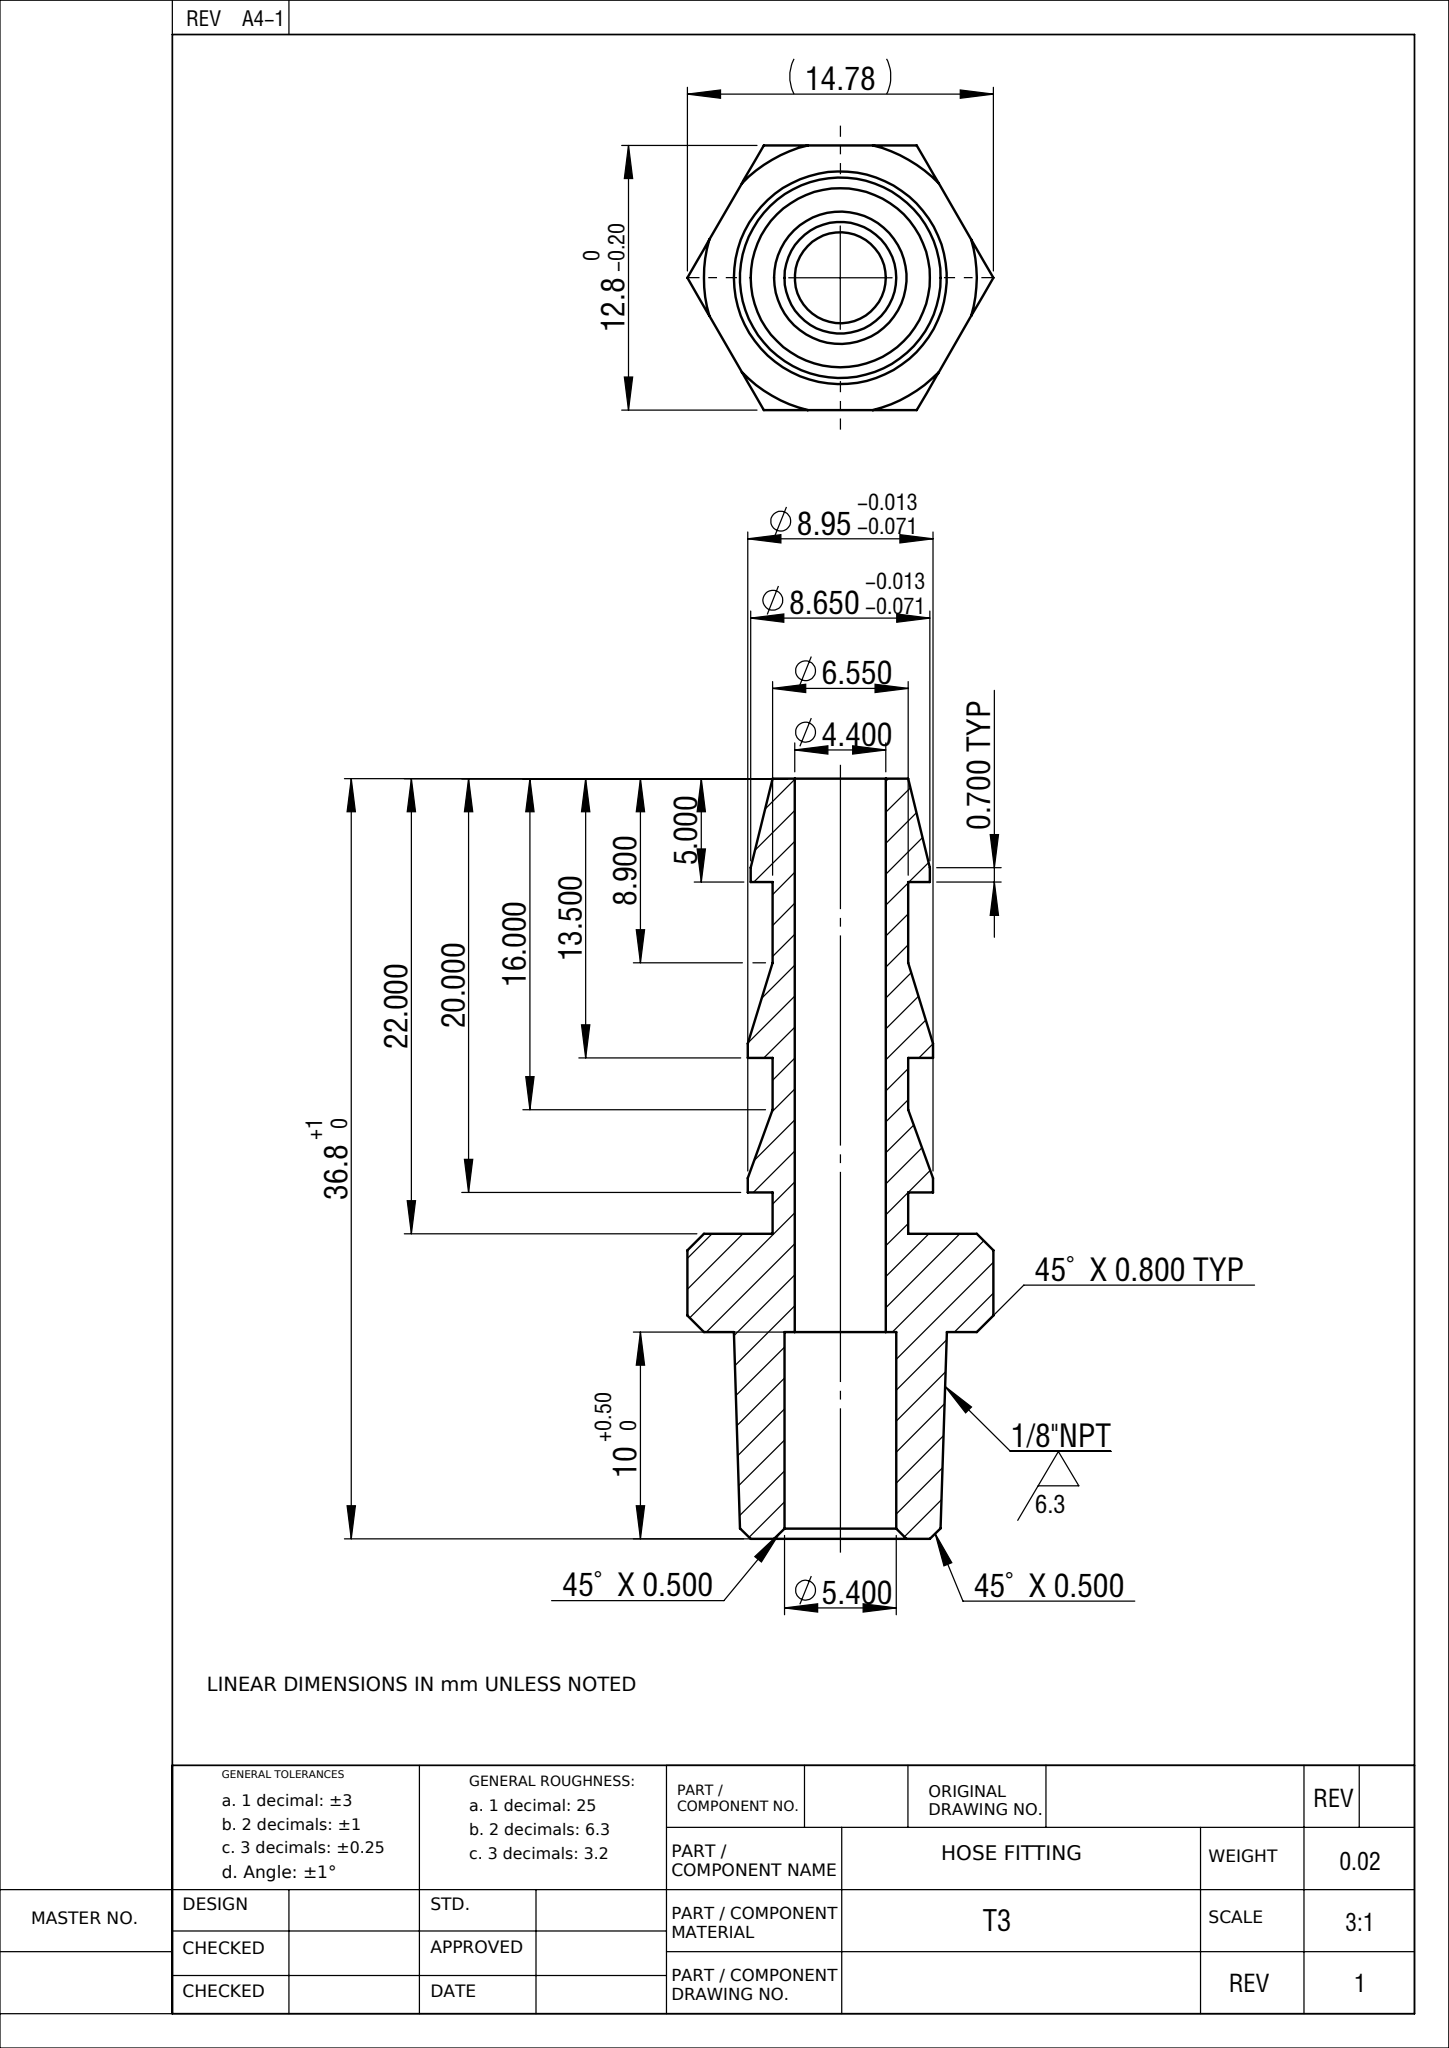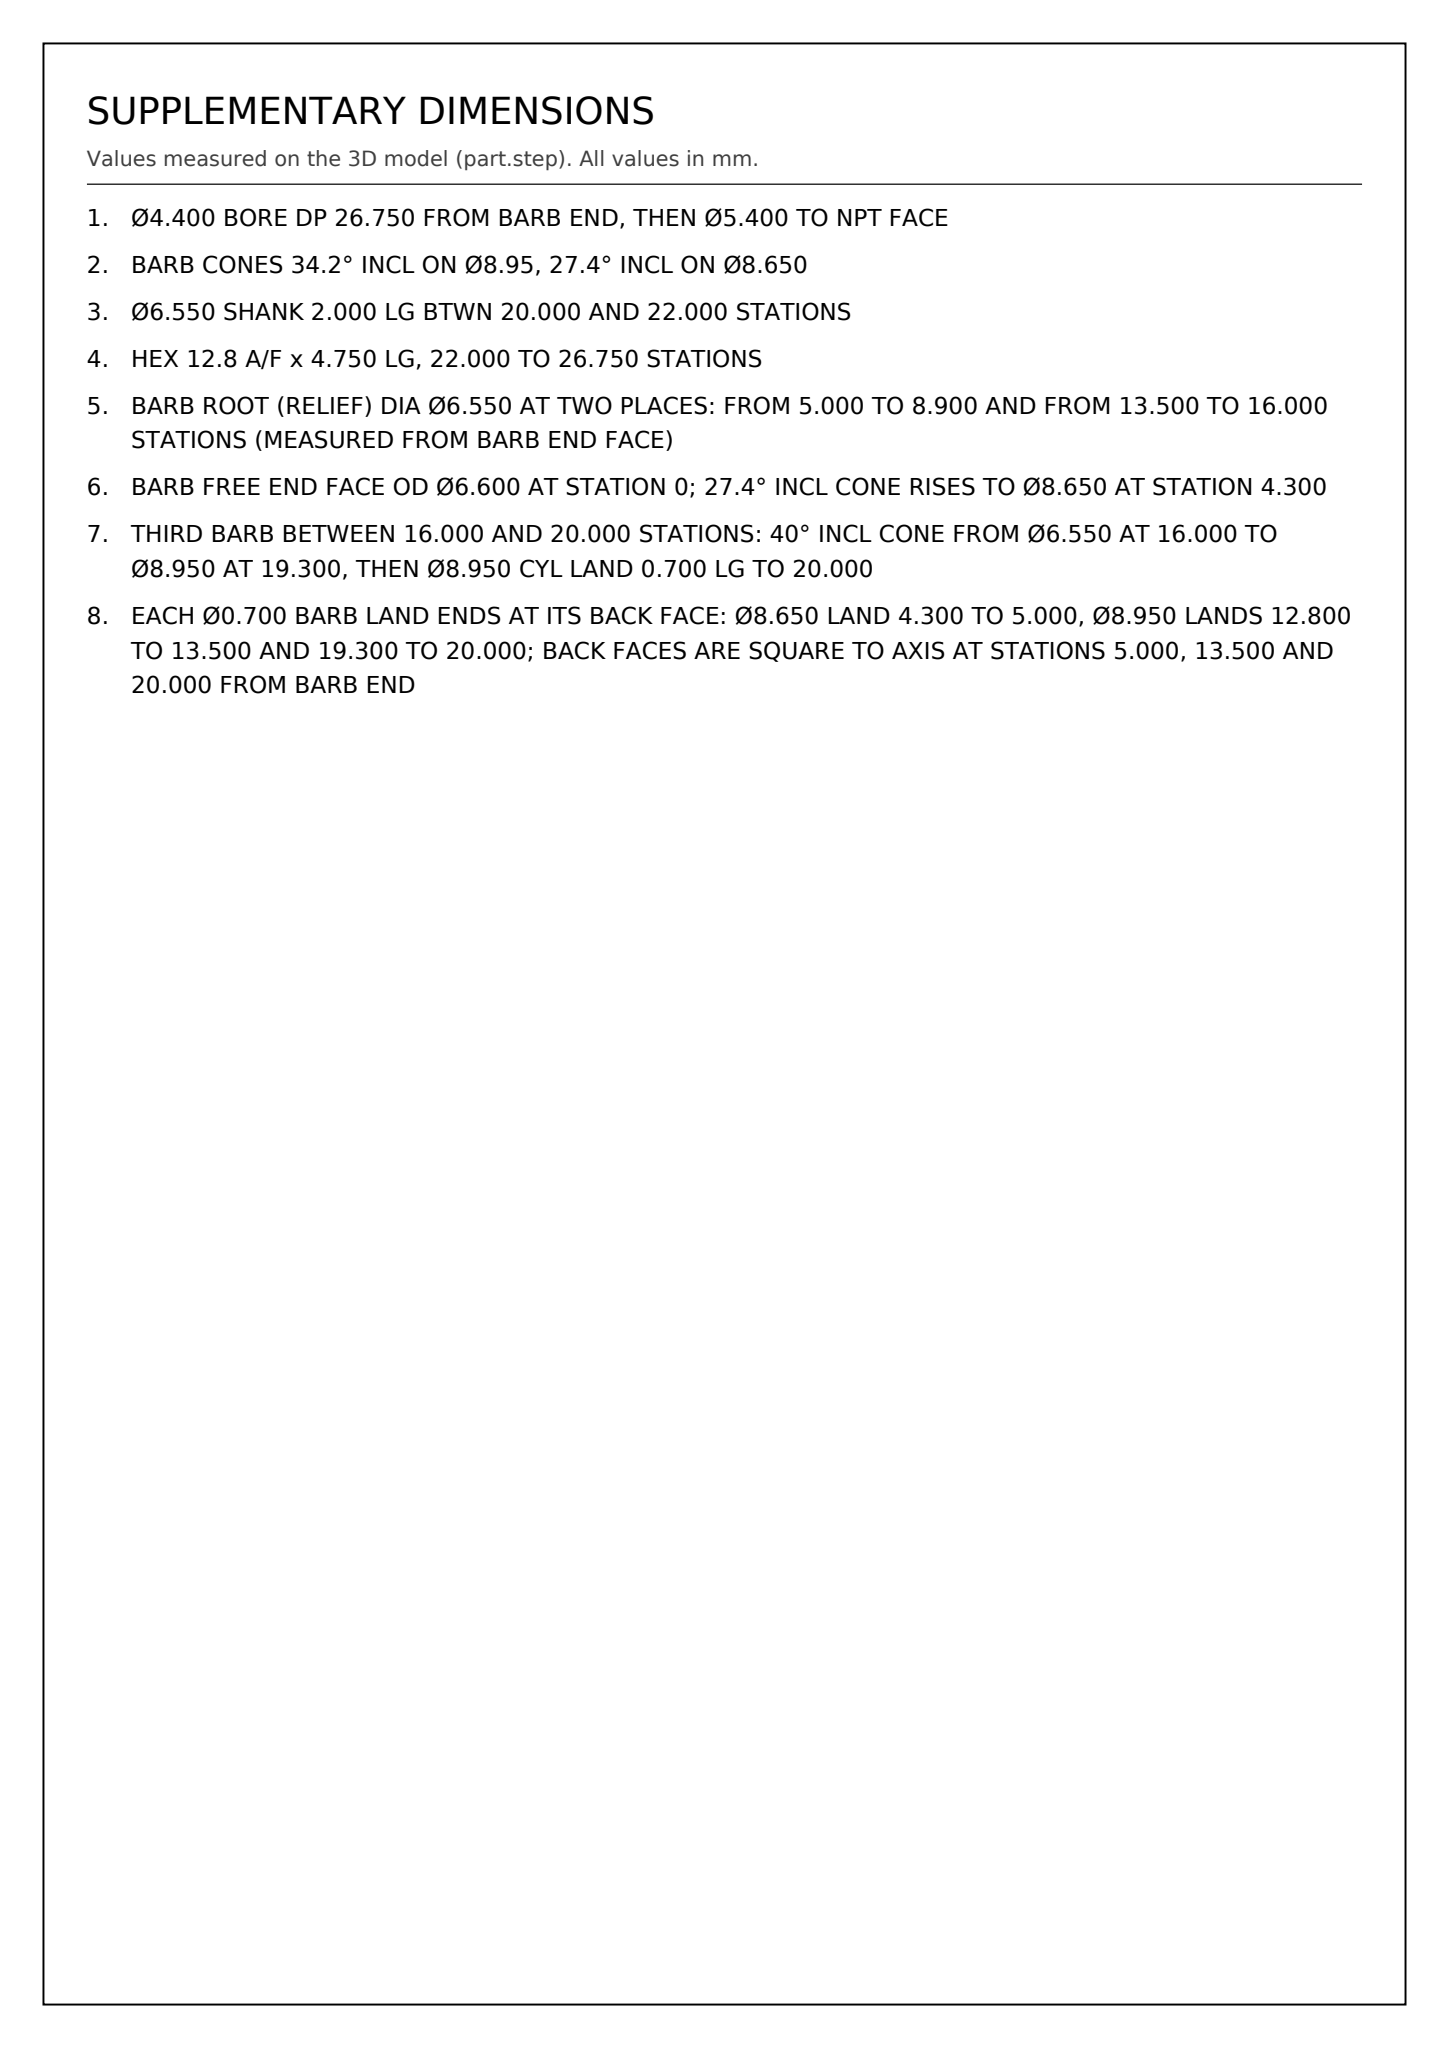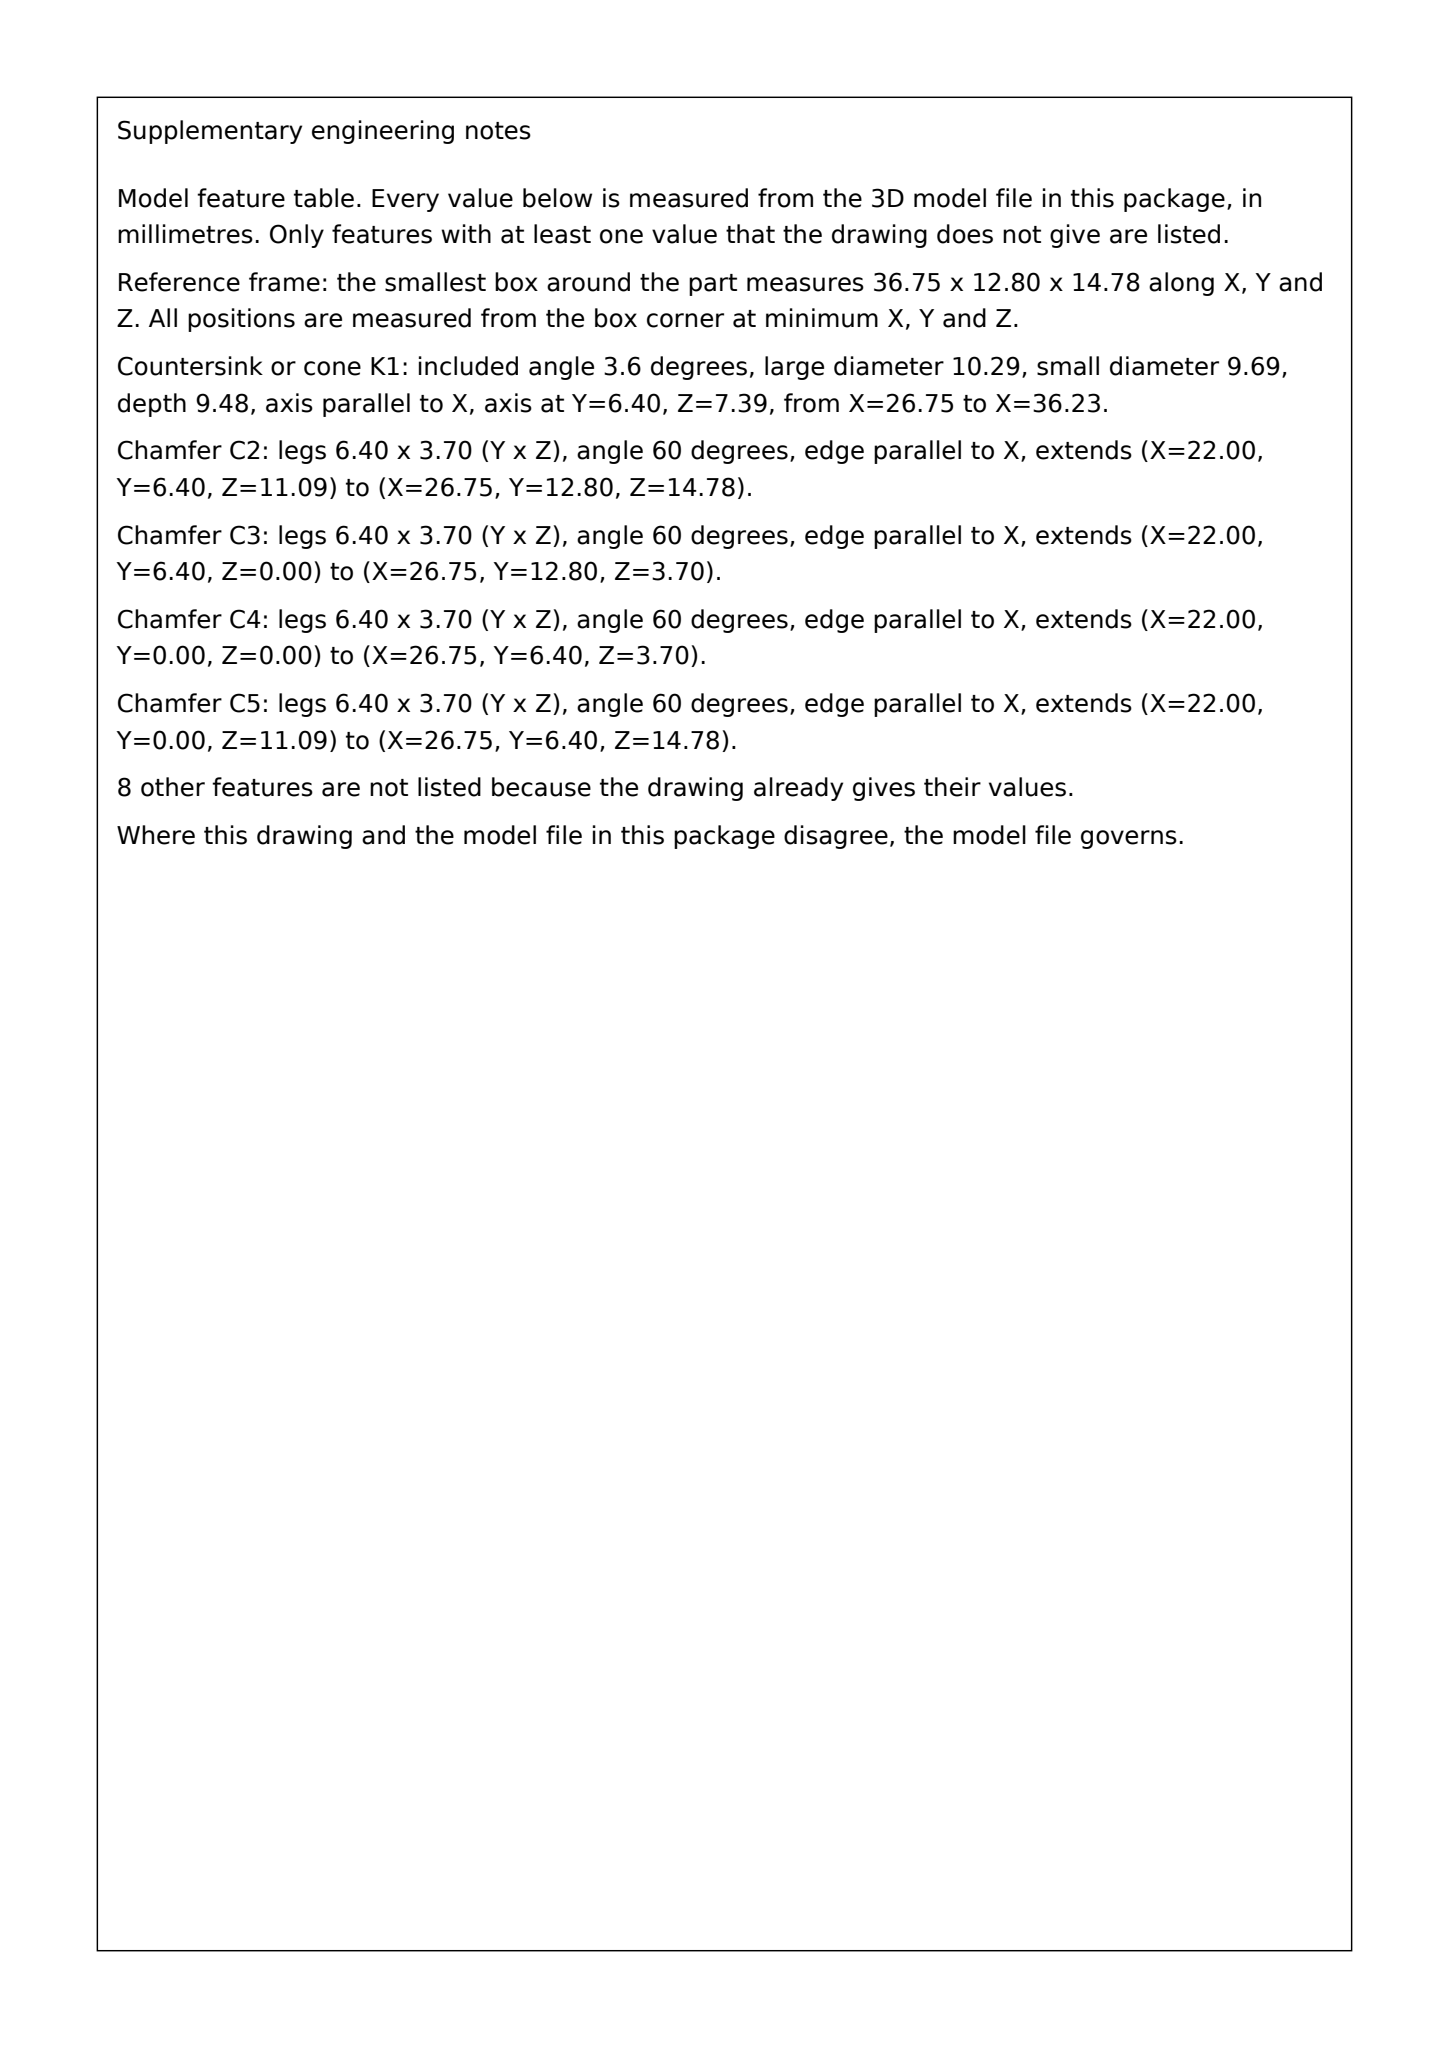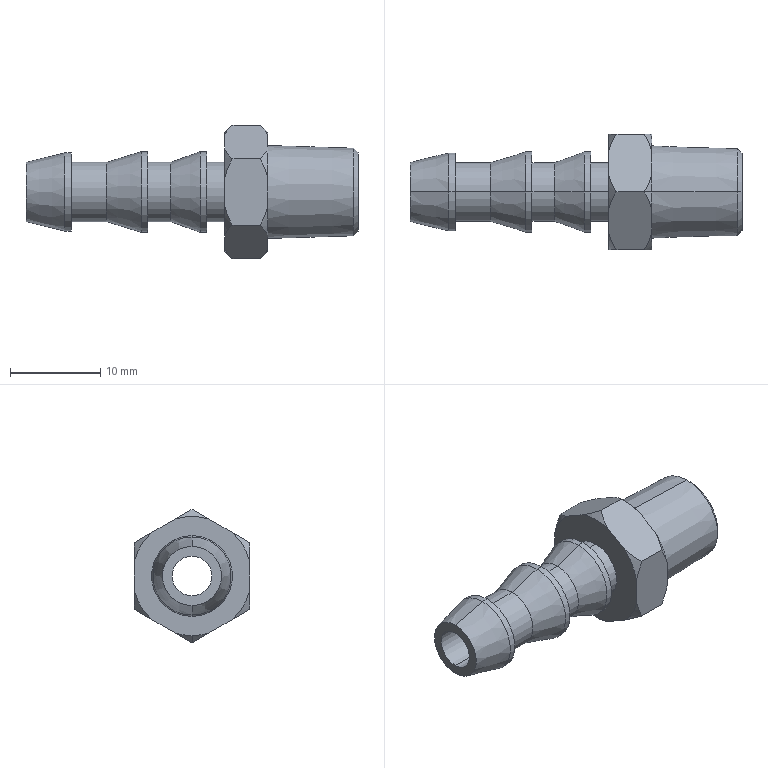Part | SolidWorks | mm | 1 solid | 56 faces | box 36.75 x 12.8 x 14.78 mm | volume 1761 mm3 | cone 26 | cylinder 16 | plane 14 | commonest cylinder face diameters 6.55 x6 8.95 x4 5.4 x2 8.65 x2 4.4 x2
Drawing notes:
Ø4.400 BORE DP 26.750 FROM BARB END, THEN Ø5.400 TO NPT FACE | from the solid: Ø4.4 cyl L=26.75 from x=0; Ø5.4 cyl L=9.5 from x=26.75 to 36.25; bbox L=36.75
BARB CONES 34.2° INCL ON Ø8.95, 27.4° INCL ON Ø8.650 | from the solid: cones [34.2, ref_dia 8.95] and [27.4, ref_dia 8.65]
Ø6.550 SHANK 2.000 LG BTWN 20.000 AND 22.000 STATIONS | from the solid: Ø6.55 cylinder L=2.0 between axis planes x=20.0 and x=22.0
HEX 12.8 A/F x 4.750 LG, 22.000 TO 26.750 STATIONS | from the solid: axis planes x=22.0 and x=26.75; 26.75 = 36.75 - 10 NPT length
BARB ROOT (RELIEF) DIA Ø6.550 AT TWO PLACES: FROM 5.000 TO 8.900 AND FROM 13.500 TO 16.000 STATIONS (MEASURED FROM BARB END FACE) | from the solid: cylinders: boss/shaft Ø6.55 x from 5.0 to 8.9; boss/shaft Ø6.55 x from 13.5 to 16.0
BARB FREE END FACE OD Ø6.600 AT STATION 0; 27.4° INCL CONE RISES TO Ø8.650 AT STATION 4.300 | from the solid: axis plane x=0.0 extent y [3.9,10.5] / z [4.1,10.7] = 6.6 annulus OD; cone 27.4° ref dia 8.65 from x 0.0, length 4.3
THIRD BARB BETWEEN 16.000 AND 20.000 STATIONS: 40° INCL CONE FROM Ø6.550 AT 16.000 TO Ø8.950 AT 19.300, THEN Ø8.950 CYL LAND 0.700 LG TO 20.000 | from the solid: cone 40.0° ref dia 8.95 bbox_from x=16.0 size x 3.3; cylinder boss/shaft Ø8.95 x from 19.3 to 20.0
EACH Ø0.700 BARB LAND ENDS AT ITS BACK FACE: Ø8.650 LAND 4.300 TO 5.000, Ø8.950 LANDS 12.800 TO 13.500 AND 19.300 TO 20.000; BACK FACES ARE SQUARE TO AXIS AT STATIONS 5.000, 13.500 AND 20.000 FROM BARB END | from the solid: cylinders Ø8.65 x 4.3-5.0, Ø8.95 x 12.8-13.5, Ø8.95 x 19.3-20.0; axis planes x=5.0, x=13.5, x=20.0
build123d program:
from build123d import *
from OCP.BRepFilletAPI import BRepFilletAPI_MakeChamfer

# Parameters (mm, degrees)
CUT_EXTRUDE1_REACH = 40.207
SKETCH2_R          = 2.2
CUT_EXTRUDE2_START = -6
CUT_EXTRUDE2_DEPTH = 6
SKETCH4_R          = 2.7
CUT_EXTRUDE3_DEPTH = 10
CHAMFER1_SIZE      = 0.5
CHAMFER1_SIZE2     = 0.5164


with BuildPart() as part:
    # Sketch1 → Revolve1 (revolve)
    with BuildSketch(Plane.XY, mode=Mode.PRIVATE) as revolve1_sk:
        Polygon((-27.85, 3.275), (-31.75, 3.275), (-31.75, 4.325), (-32.45, 4.325), (-36.75, 3.275), (-36.75, 0), (0, 0), (0, 4.831), (-10, 5.144), (-10, 7.39), (-14.75, 7.39), (-14.75, 3.275), (-16.75, 3.275), (-16.75, 4.475), (-17.45, 4.475), (-20.75, 3.275), (-23.25, 3.275), (-23.25, 4.475), (-23.95, 4.475), align=None)
    revolve(revolve1_sk.sketch.rotate(Axis((-78.266, 0, 0), (1, 0, 0)), 90), axis=Axis((-78.266, 0, 0), (1, 0, 0)))

    # Sketch2 → Cut-Extrude1 (cut, up to next)
    with BuildSketch(Plane(origin=(0, 0, 0), x_dir=(0, 0, -1), z_dir=(1, 0, 0)), mode=Mode.PRIVATE) as cut_extrude1_sk1:
        Circle(SKETCH2_R)
    cut_extrude1_tool1 = extrude(cut_extrude1_sk1.sketch, amount=-CUT_EXTRUDE1_REACH, mode=Mode.PRIVATE) & part.part
    add(cut_extrude1_tool1.solids().sort_by_distance((0, 0, 0))[0], mode=Mode.SUBTRACT)

    # Sketch3 → Cut-Extrude2 (cut)
    with BuildSketch(Plane(origin=(-10, 0, 0), x_dir=(0, 0, -1), z_dir=(1, 0, 0)).offset(CUT_EXTRUDE2_START)):
        with BuildLine():
            Line((-7.39, 0), (-3.695, 6.4))
            ThreePointArc((-3.695, 6.4), (-6.4, 3.695), (-7.39, 0))
        make_face()
        with BuildLine():
            ThreePointArc((3.695, 6.4), (0, 7.39), (-3.695, 6.4))
            Line((-3.695, 6.4), (3.695, 6.4))
        make_face()
        with BuildLine():
            ThreePointArc((7.39, 0), (6.4, 3.695), (3.695, 6.4))
            Line((3.695, 6.4), (7.39, 0))
        make_face()
        with BuildLine():
            ThreePointArc((3.695, -6.4), (6.4, -3.695), (7.39, 0))
            Line((7.39, 0), (3.695, -6.4))
        make_face()
        with BuildLine():
            Line((3.695, -6.4), (-3.695, -6.4))
            ThreePointArc((-3.695, -6.4), (0, -7.39), (3.695, -6.4))
        make_face()
        with BuildLine():
            Line((-3.695, -6.4), (-7.39, 0))
            ThreePointArc((-7.39, 0), (-6.4, -3.695), (-3.695, -6.4))
        make_face()
    extrude(amount=CUT_EXTRUDE2_DEPTH, mode=Mode.SUBTRACT)

    # Sketch4 → Cut-Extrude3 (cut)
    with BuildSketch(Plane(origin=(0, 0, 0), x_dir=(0, 0, -1), z_dir=(1, 0, 0))):
        Circle(SKETCH4_R)
    extrude(amount=-CUT_EXTRUDE3_DEPTH, mode=Mode.SUBTRACT)

    # Chamfer1: one chamfer whose edges measure the first distance from different faces: ONE call of the kernel's chamfer builder (chamfer() names one face for all edges)
    chamfer1_edges_1 = [part.edges().sort_by_distance(p)[0] for p in [
        (0, 0, -4.831),
    ]]
    chamfer1_side_1 = [part.faces().sort_by_distance(p)[0] for p in [
        (0, 0, -4.694),
    ]]
    chamfer1_edges_2 = [part.edges().sort_by_distance(p)[0] for p in [
        (0, 0, 2.7),
    ]]
    chamfer1 = BRepFilletAPI_MakeChamfer(part.part.solid().wrapped)
    for e in chamfer1_edges_1:
        chamfer1.Add(CHAMFER1_SIZE, CHAMFER1_SIZE2, e.wrapped, chamfer1_side_1[0].wrapped)  # the first distance lies on this face
    for e in chamfer1_edges_2:
        chamfer1.Add(CHAMFER1_SIZE, e.wrapped)
    add(Compound.cast(chamfer1.Shape()), mode=Mode.REPLACE)

    # Sketch5 → Cut-Revolve3 (revolve, cut)
    with BuildSketch(Plane(origin=(0, 0, 0), x_dir=(1, 0, 0), z_dir=(0, 1, 0)), mode=Mode.PRIVATE) as cut_revolve3_sk:
        Polygon((-13.95, 7.39), (-14.75, 6.59), (-14.75, 7.39), align=None)
        Polygon((-10, 7.39), (-10.8, 7.39), (-10, 6.59), align=None)
    revolve(cut_revolve3_sk.sketch.rotate(Axis((-36.75, 0, 0), (1, 0, 0)), 180), axis=Axis((-36.75, 0, 0), (1, 0, 0)), mode=Mode.SUBTRACT)


solid = part.part